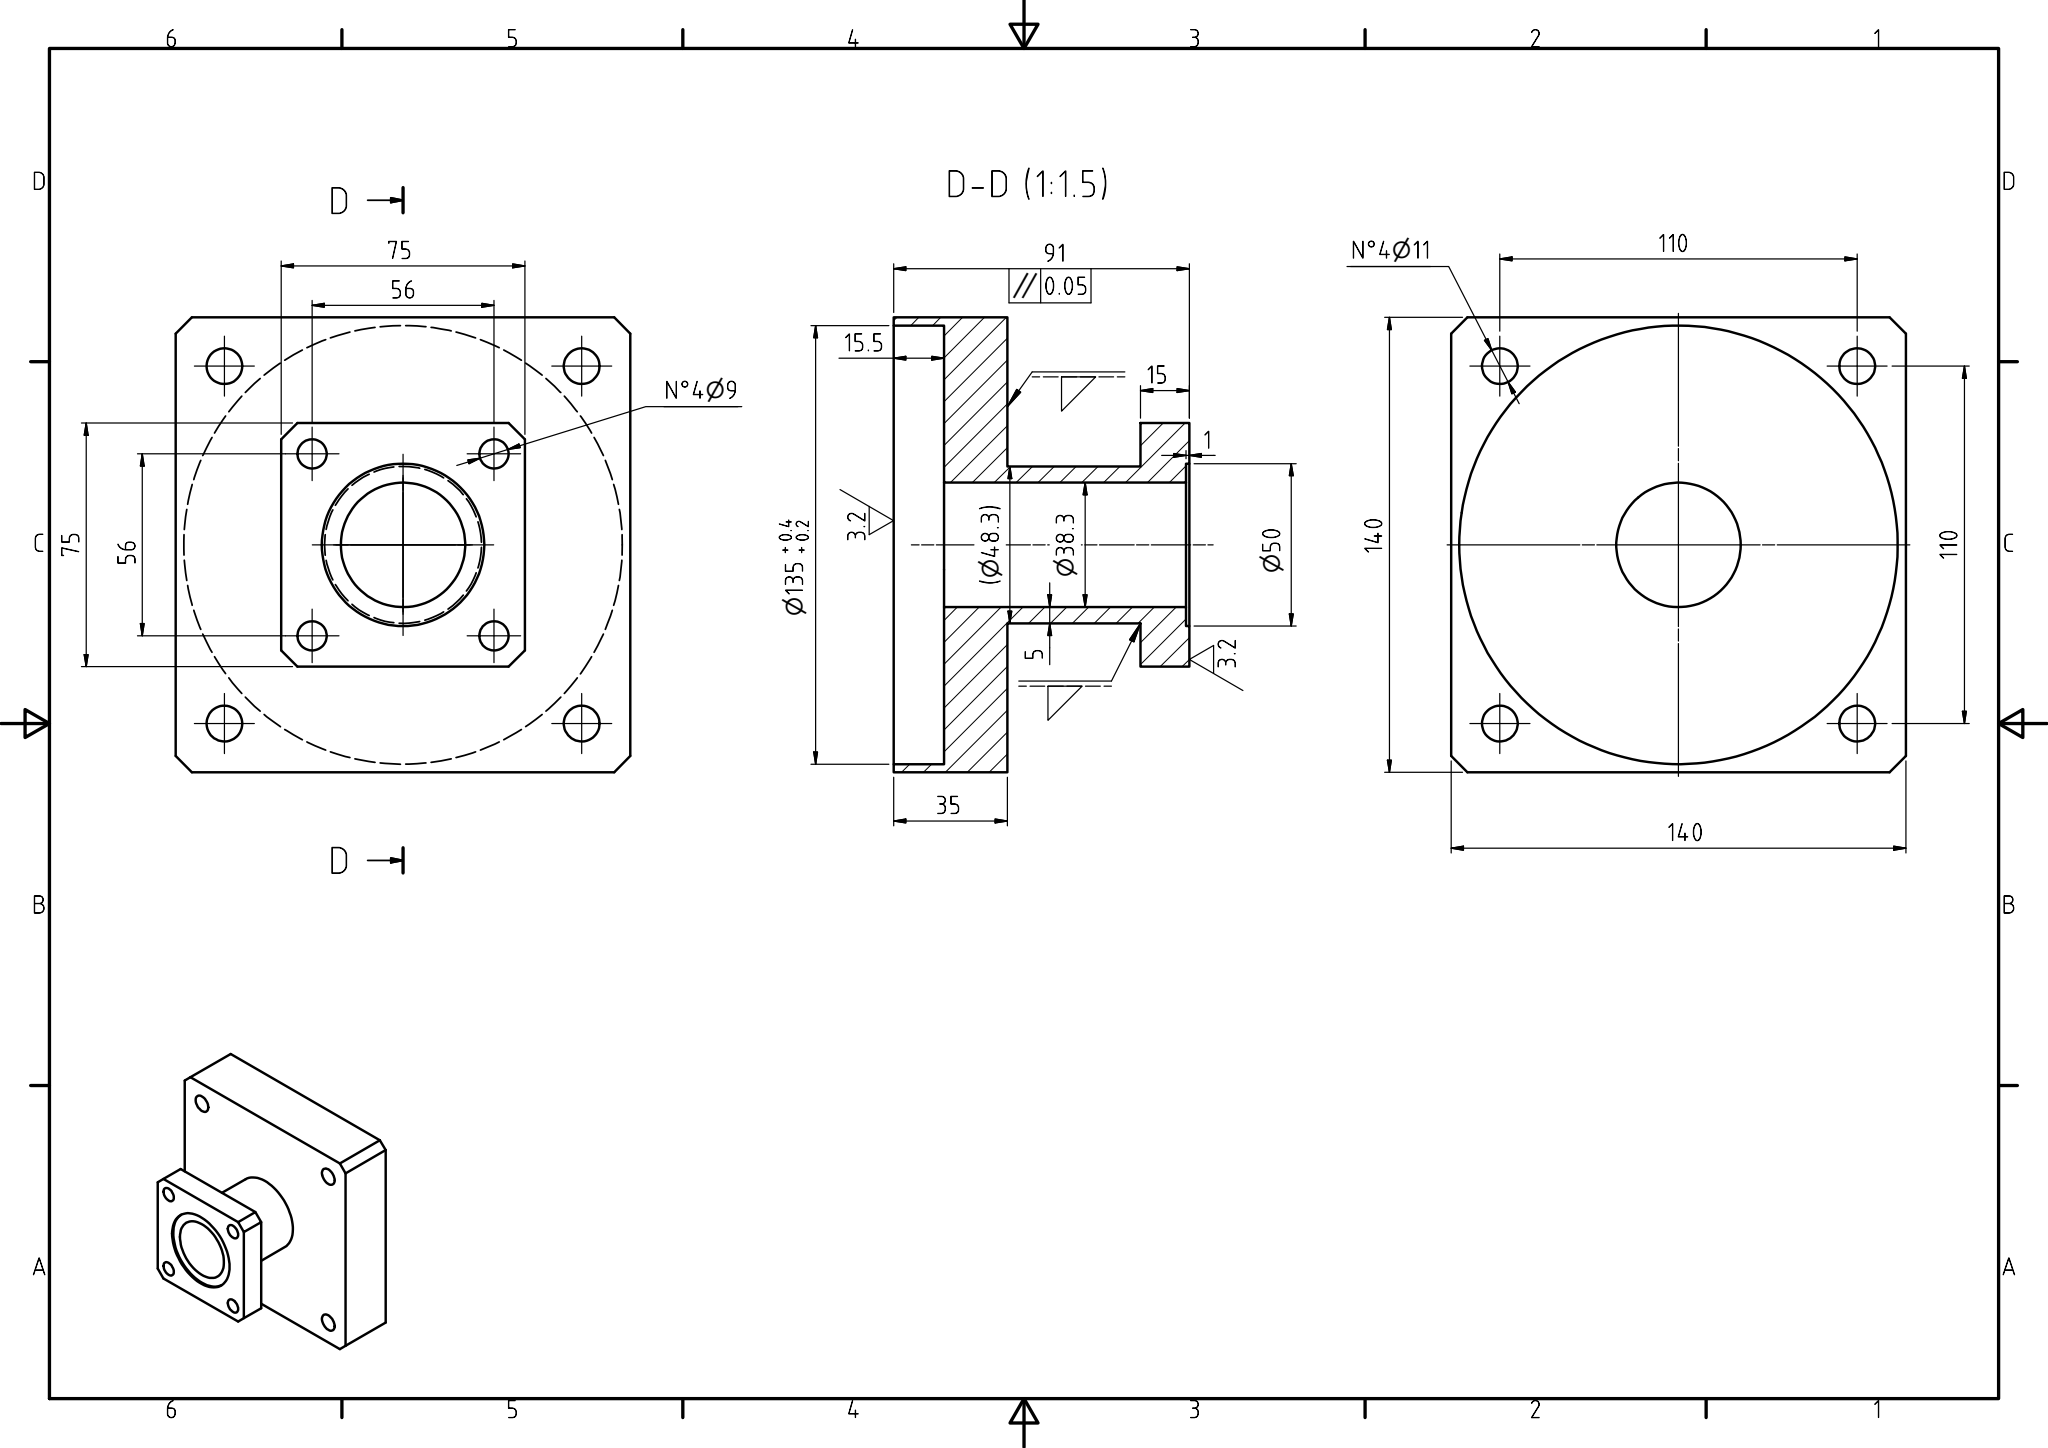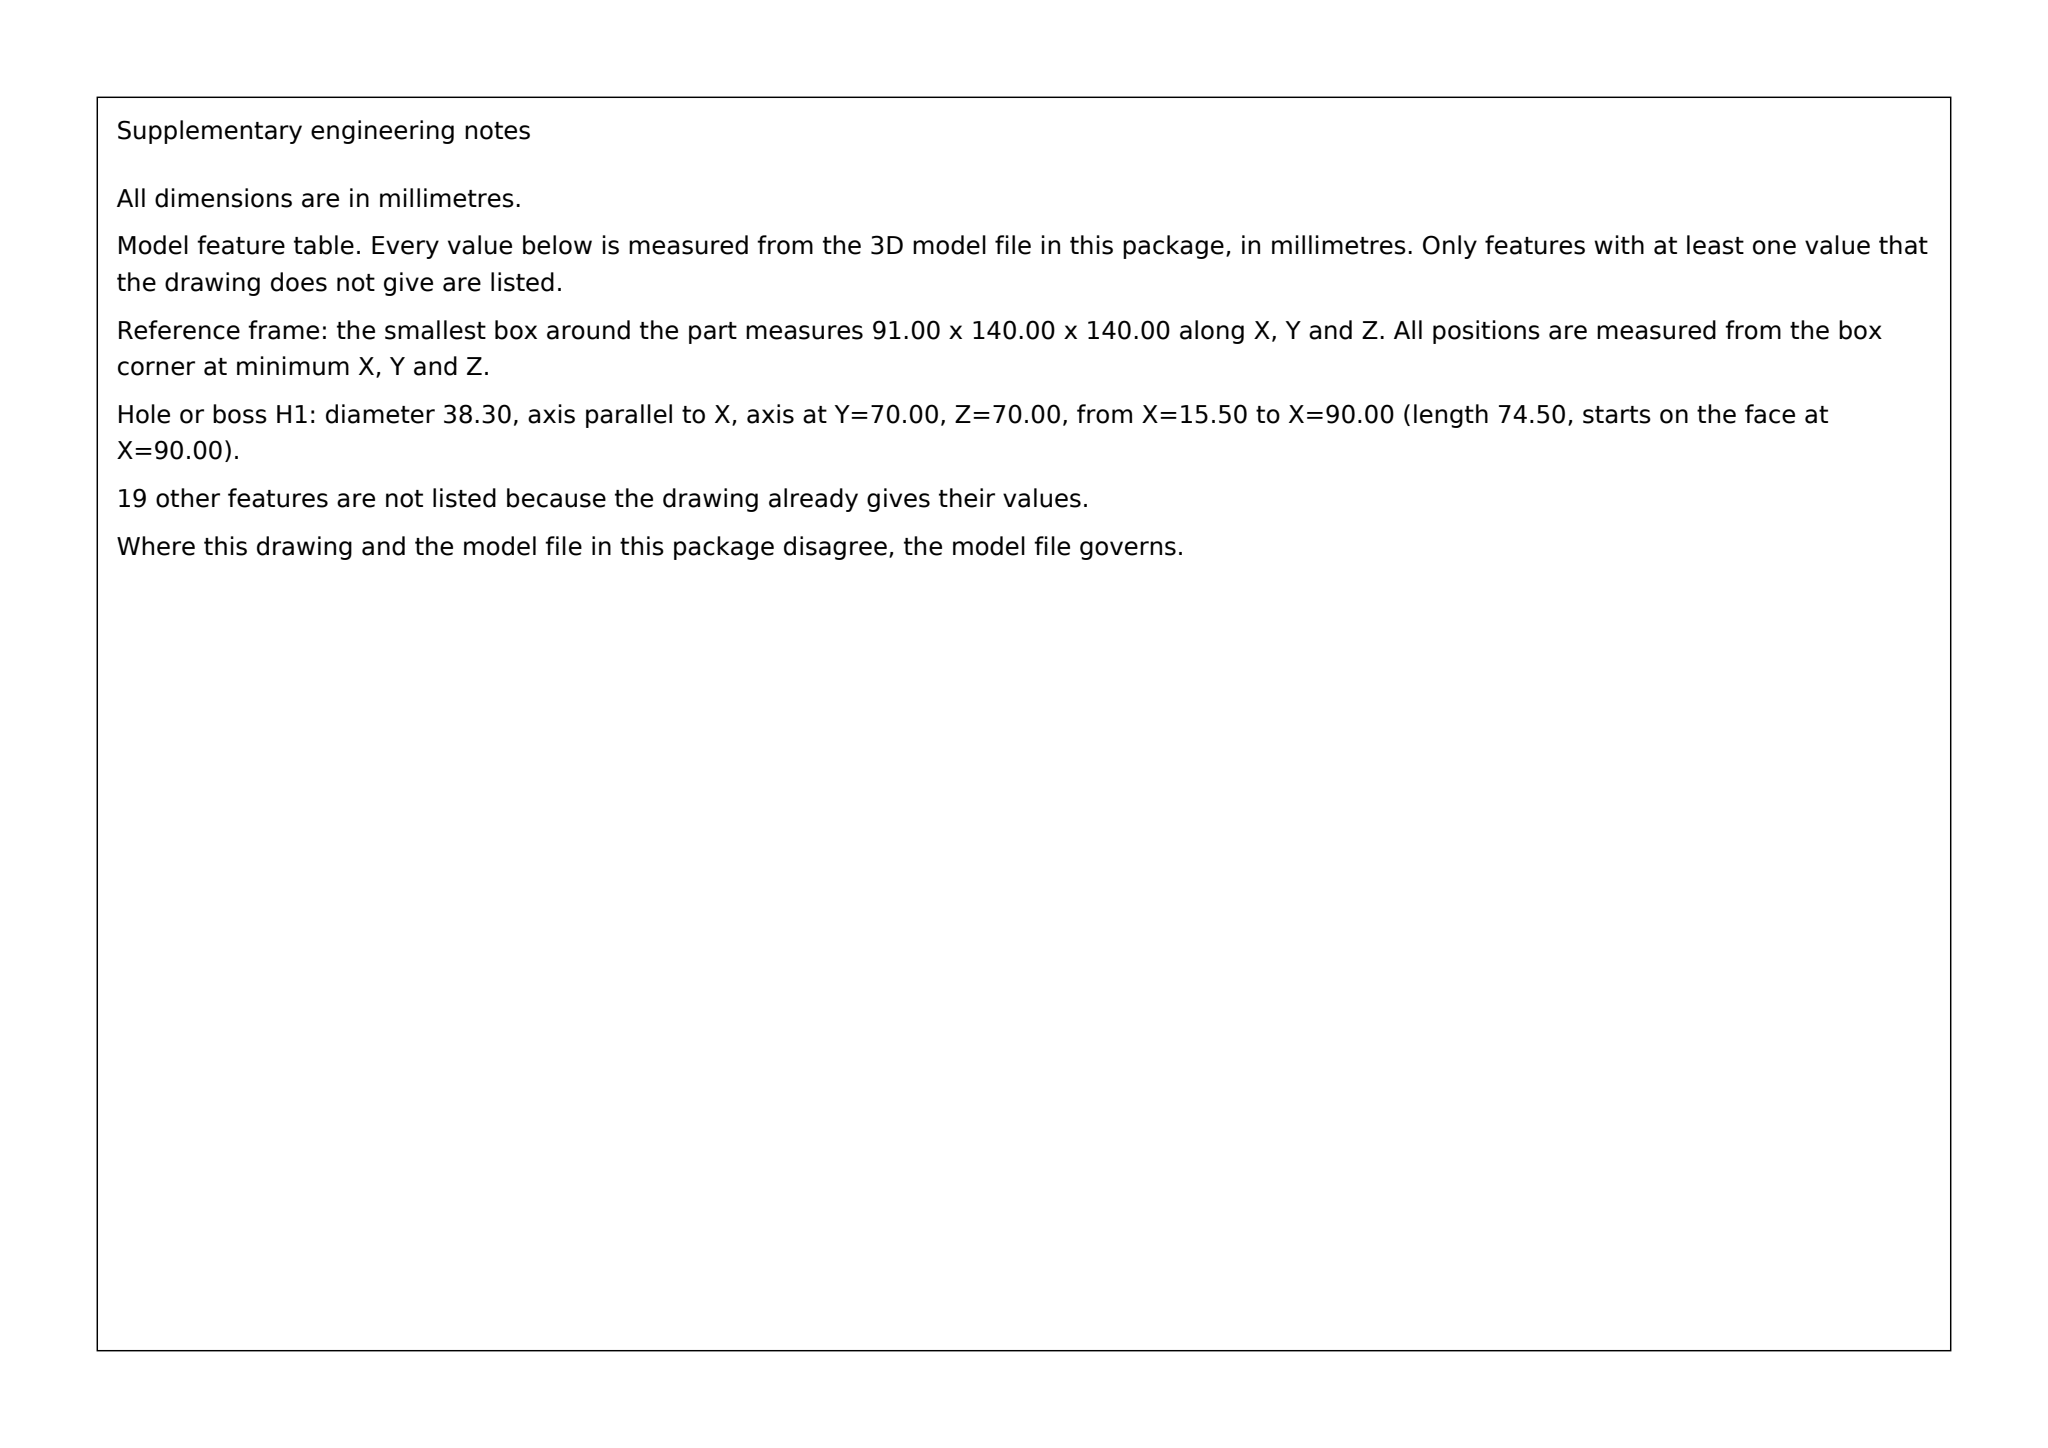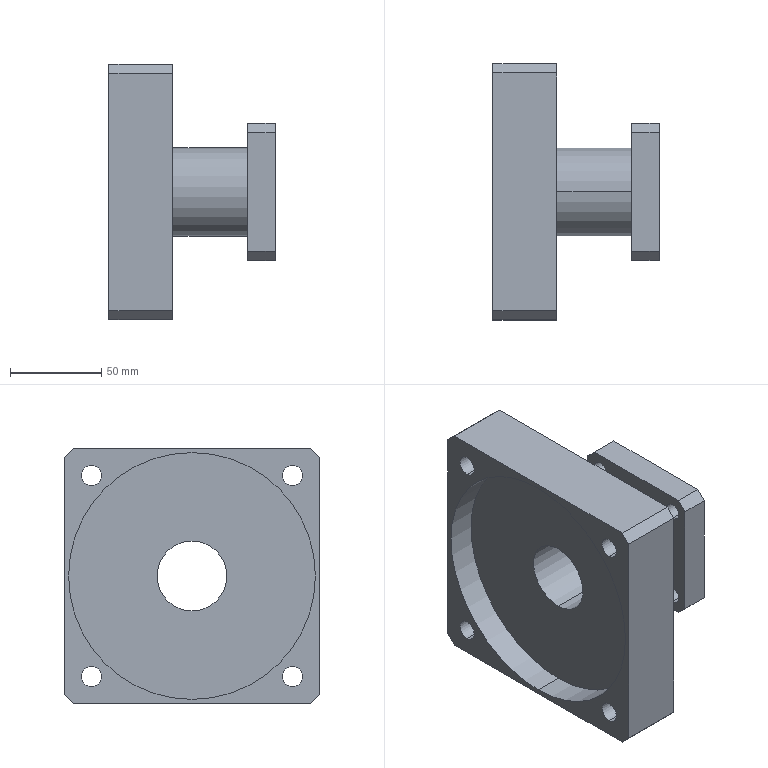Part | SolidWorks | mm | 1 solid | 46 faces | box 91 x 140 x 140 mm | volume 516216 mm3 | cylinder 24 | plane 22 | commonest cylinder face diameters 9 x8 11 x8 48.3 x2 38.3 x2 50 x2 135 x2